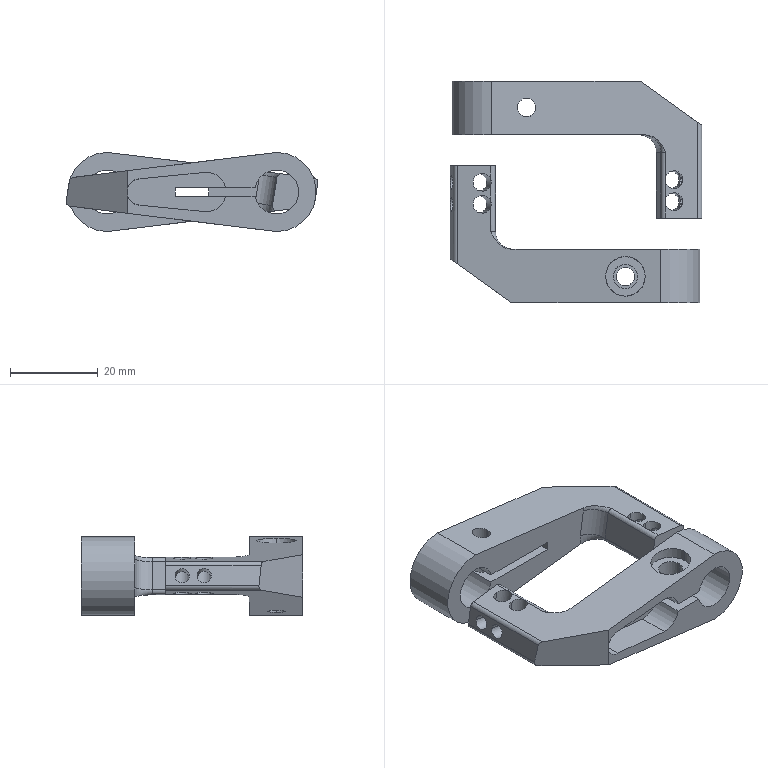CAM job | Mastercam | mm | 1 operations | part box 68.65 x 50.4 x 18
1. Contour (Ramp) | 1 - 6 平铣刀